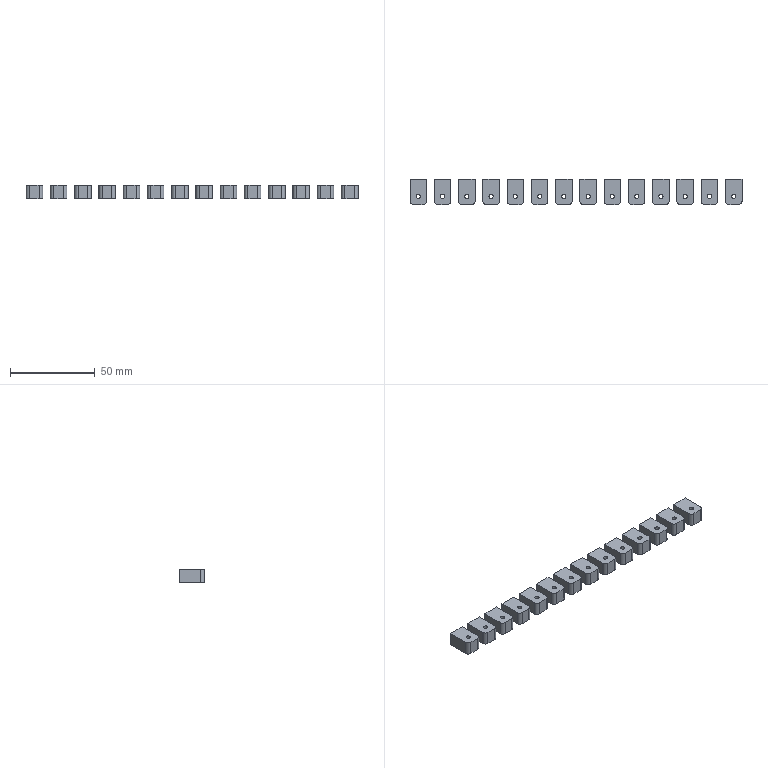CAM job | Mastercam | mm | 8 operations | part box 195.7 x 14.8 x 8
1. Facing | 24 - 100 平铣刀
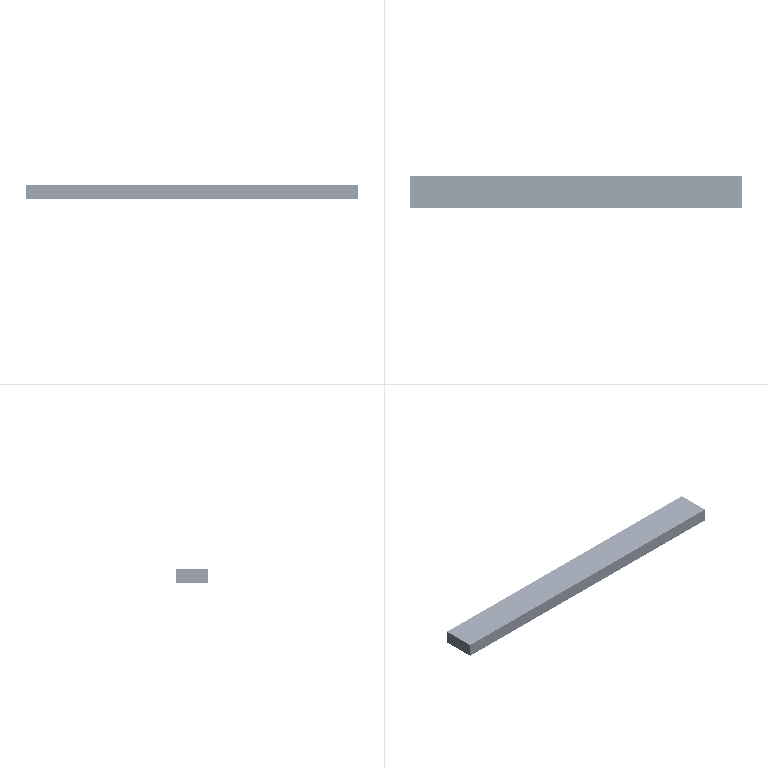2. Contour (Ramp) | 4 - 4 平铣刀
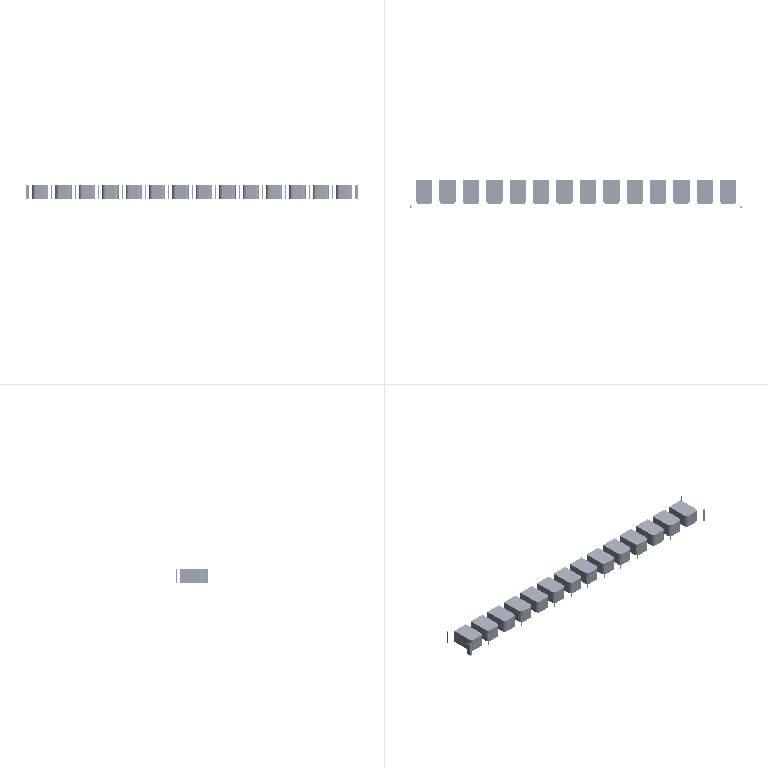3. Contour (Ramp) | 4 - 4 平铣刀
4. Contour (2D chamfer) | 7 - 4 倒角刀
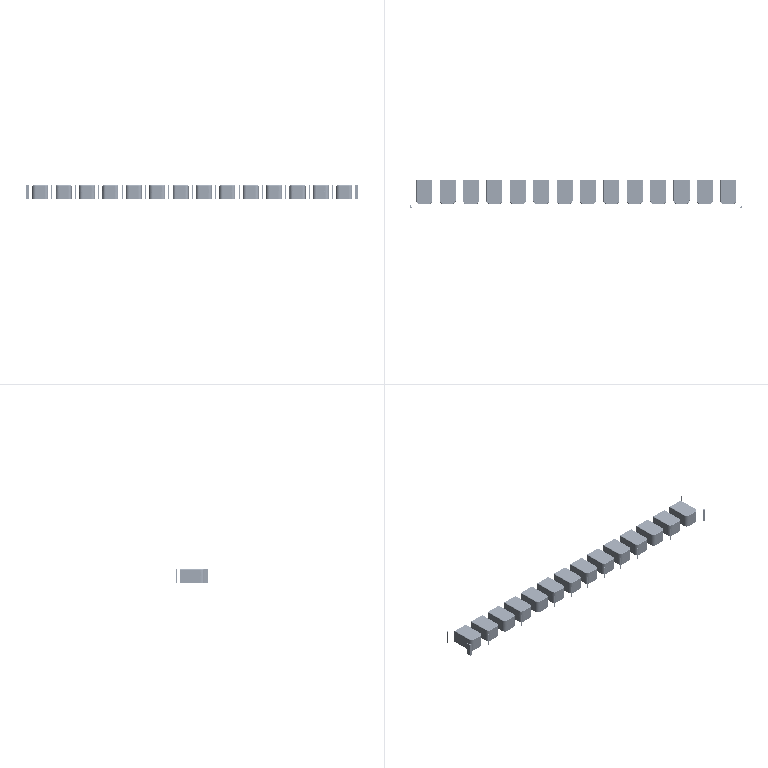5. Drill/Counterbore | 7 - 4 倒角刀
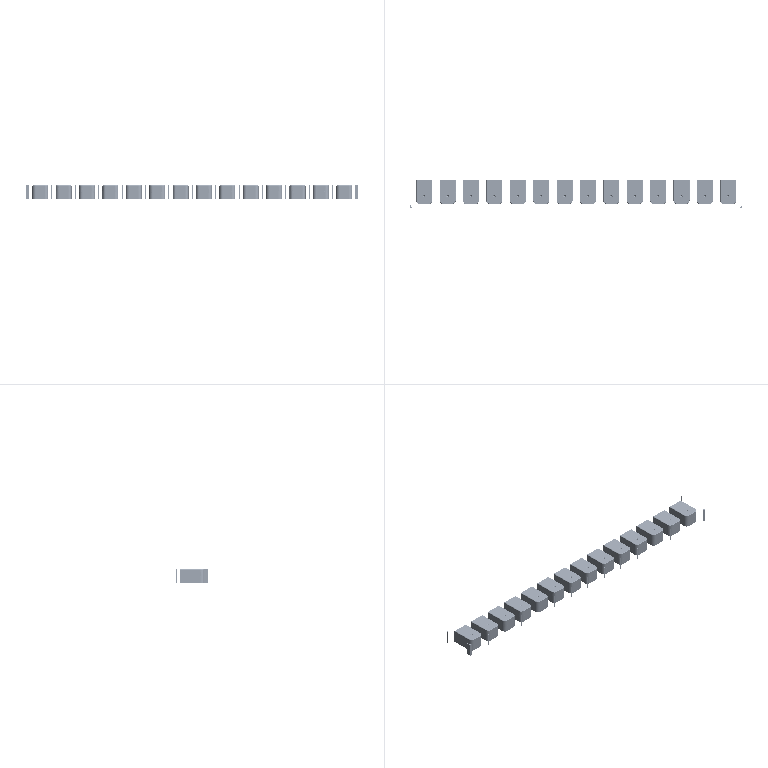6. Drill/Counterbore | 7 - 4 倒角刀
7. Facing | 12 - 12 平铣刀
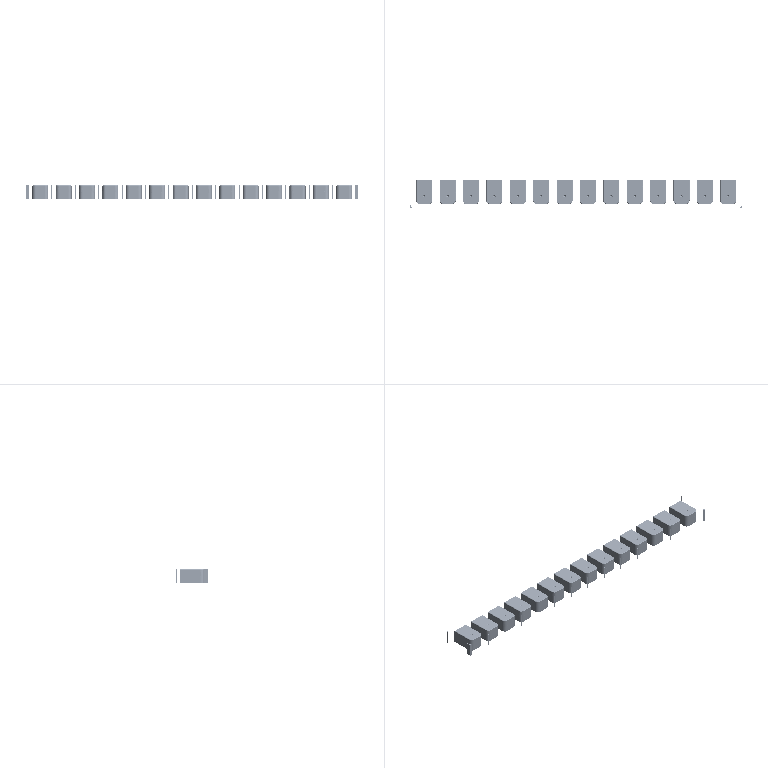8. Contour (2D chamfer) | 7 - 4 倒角刀